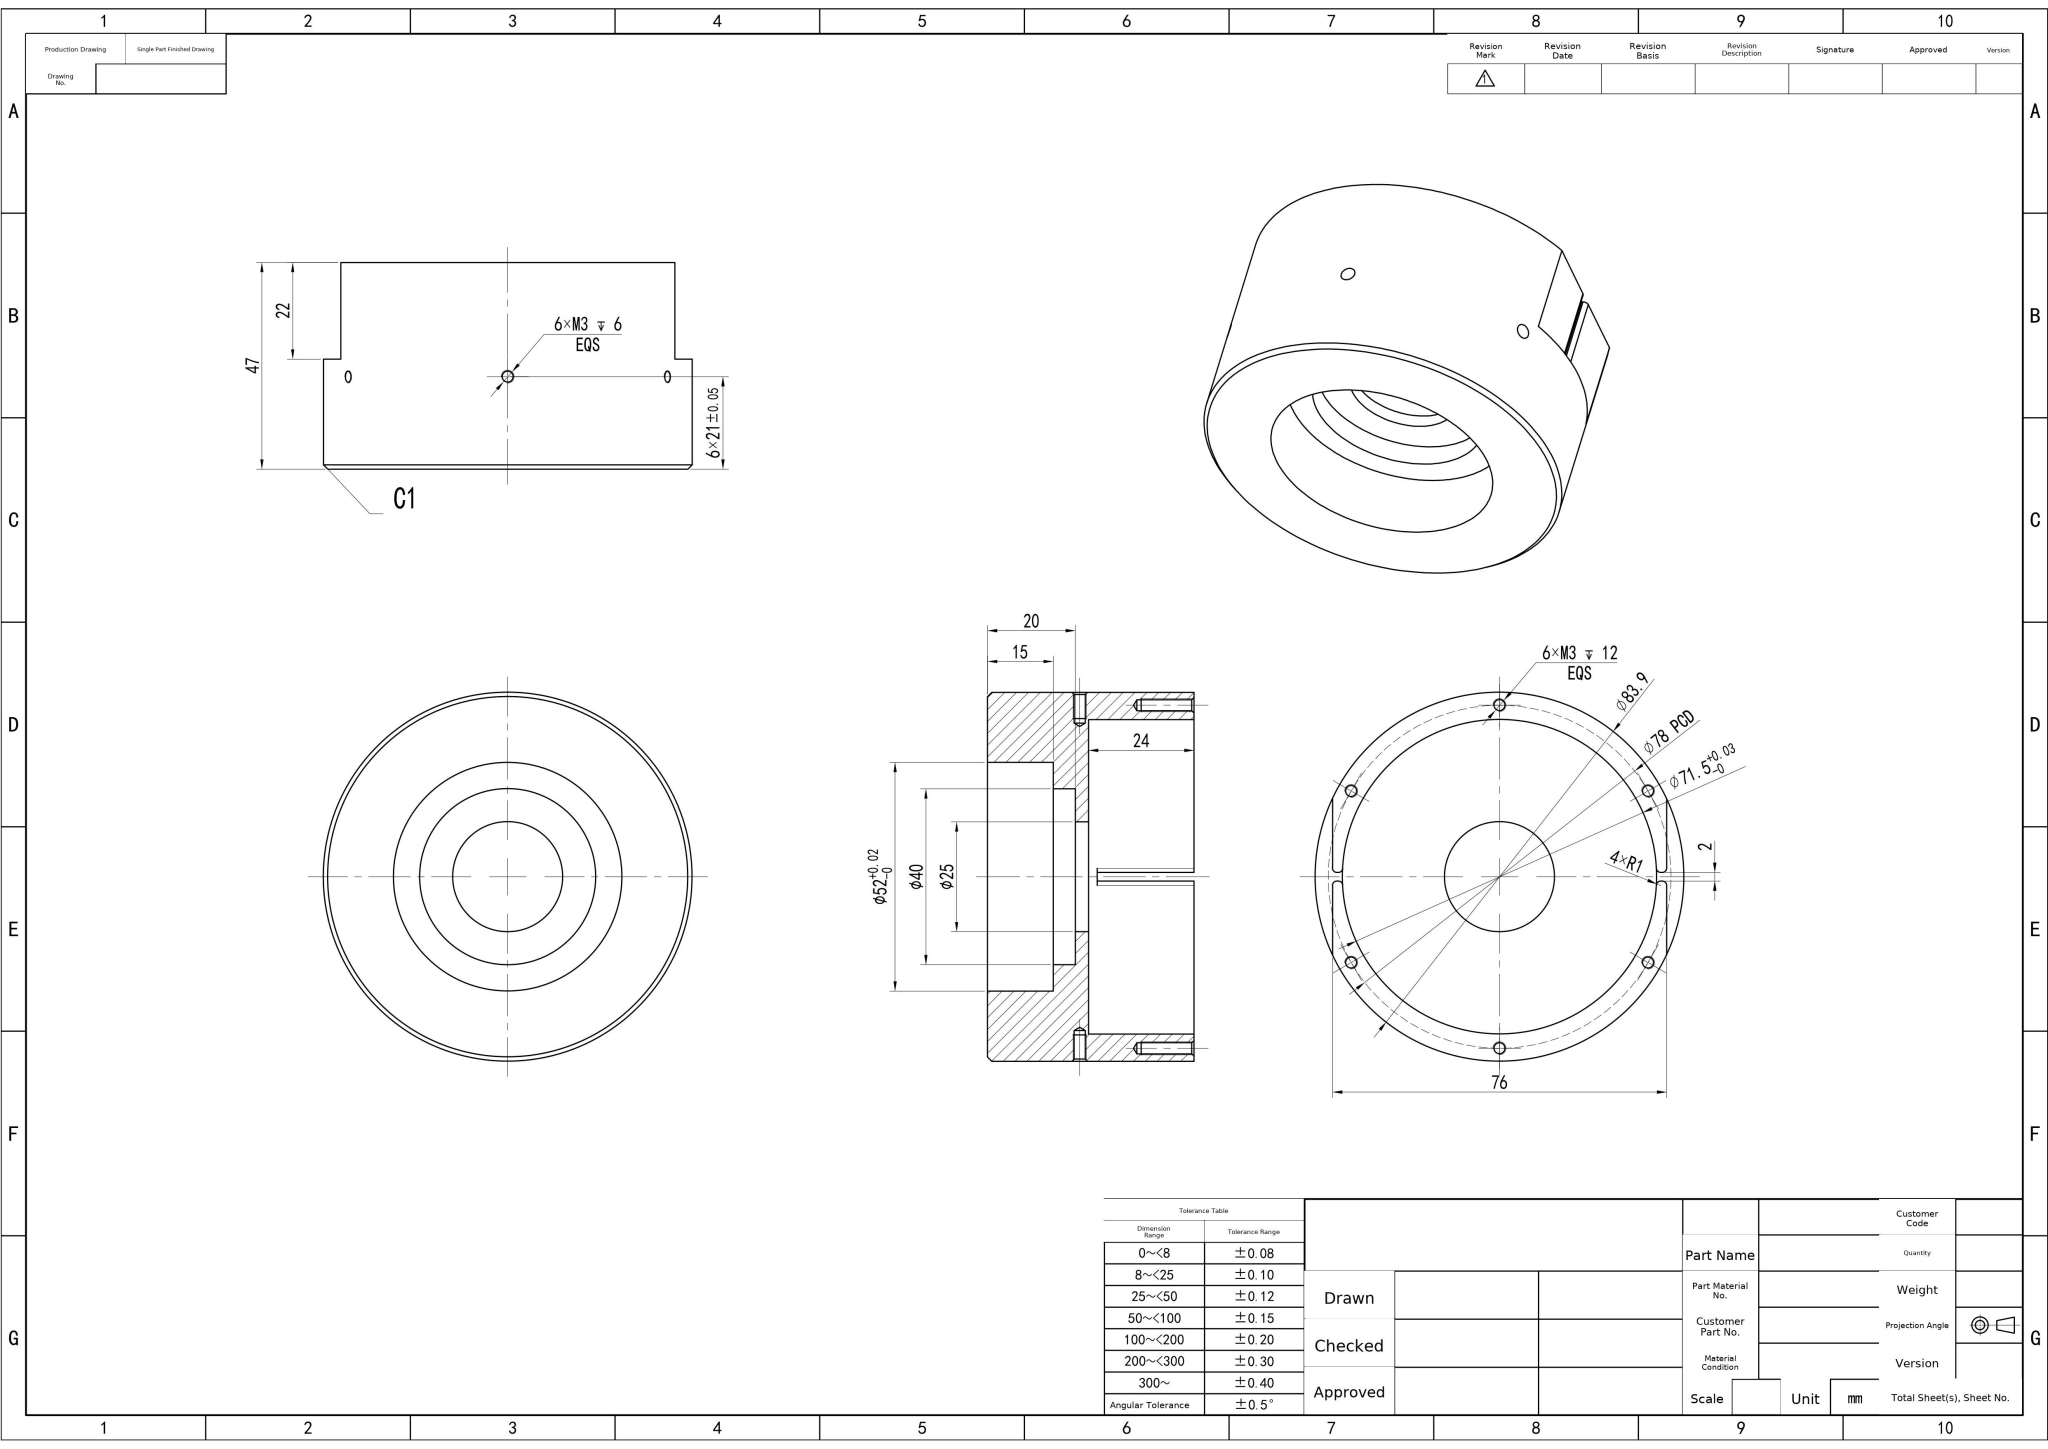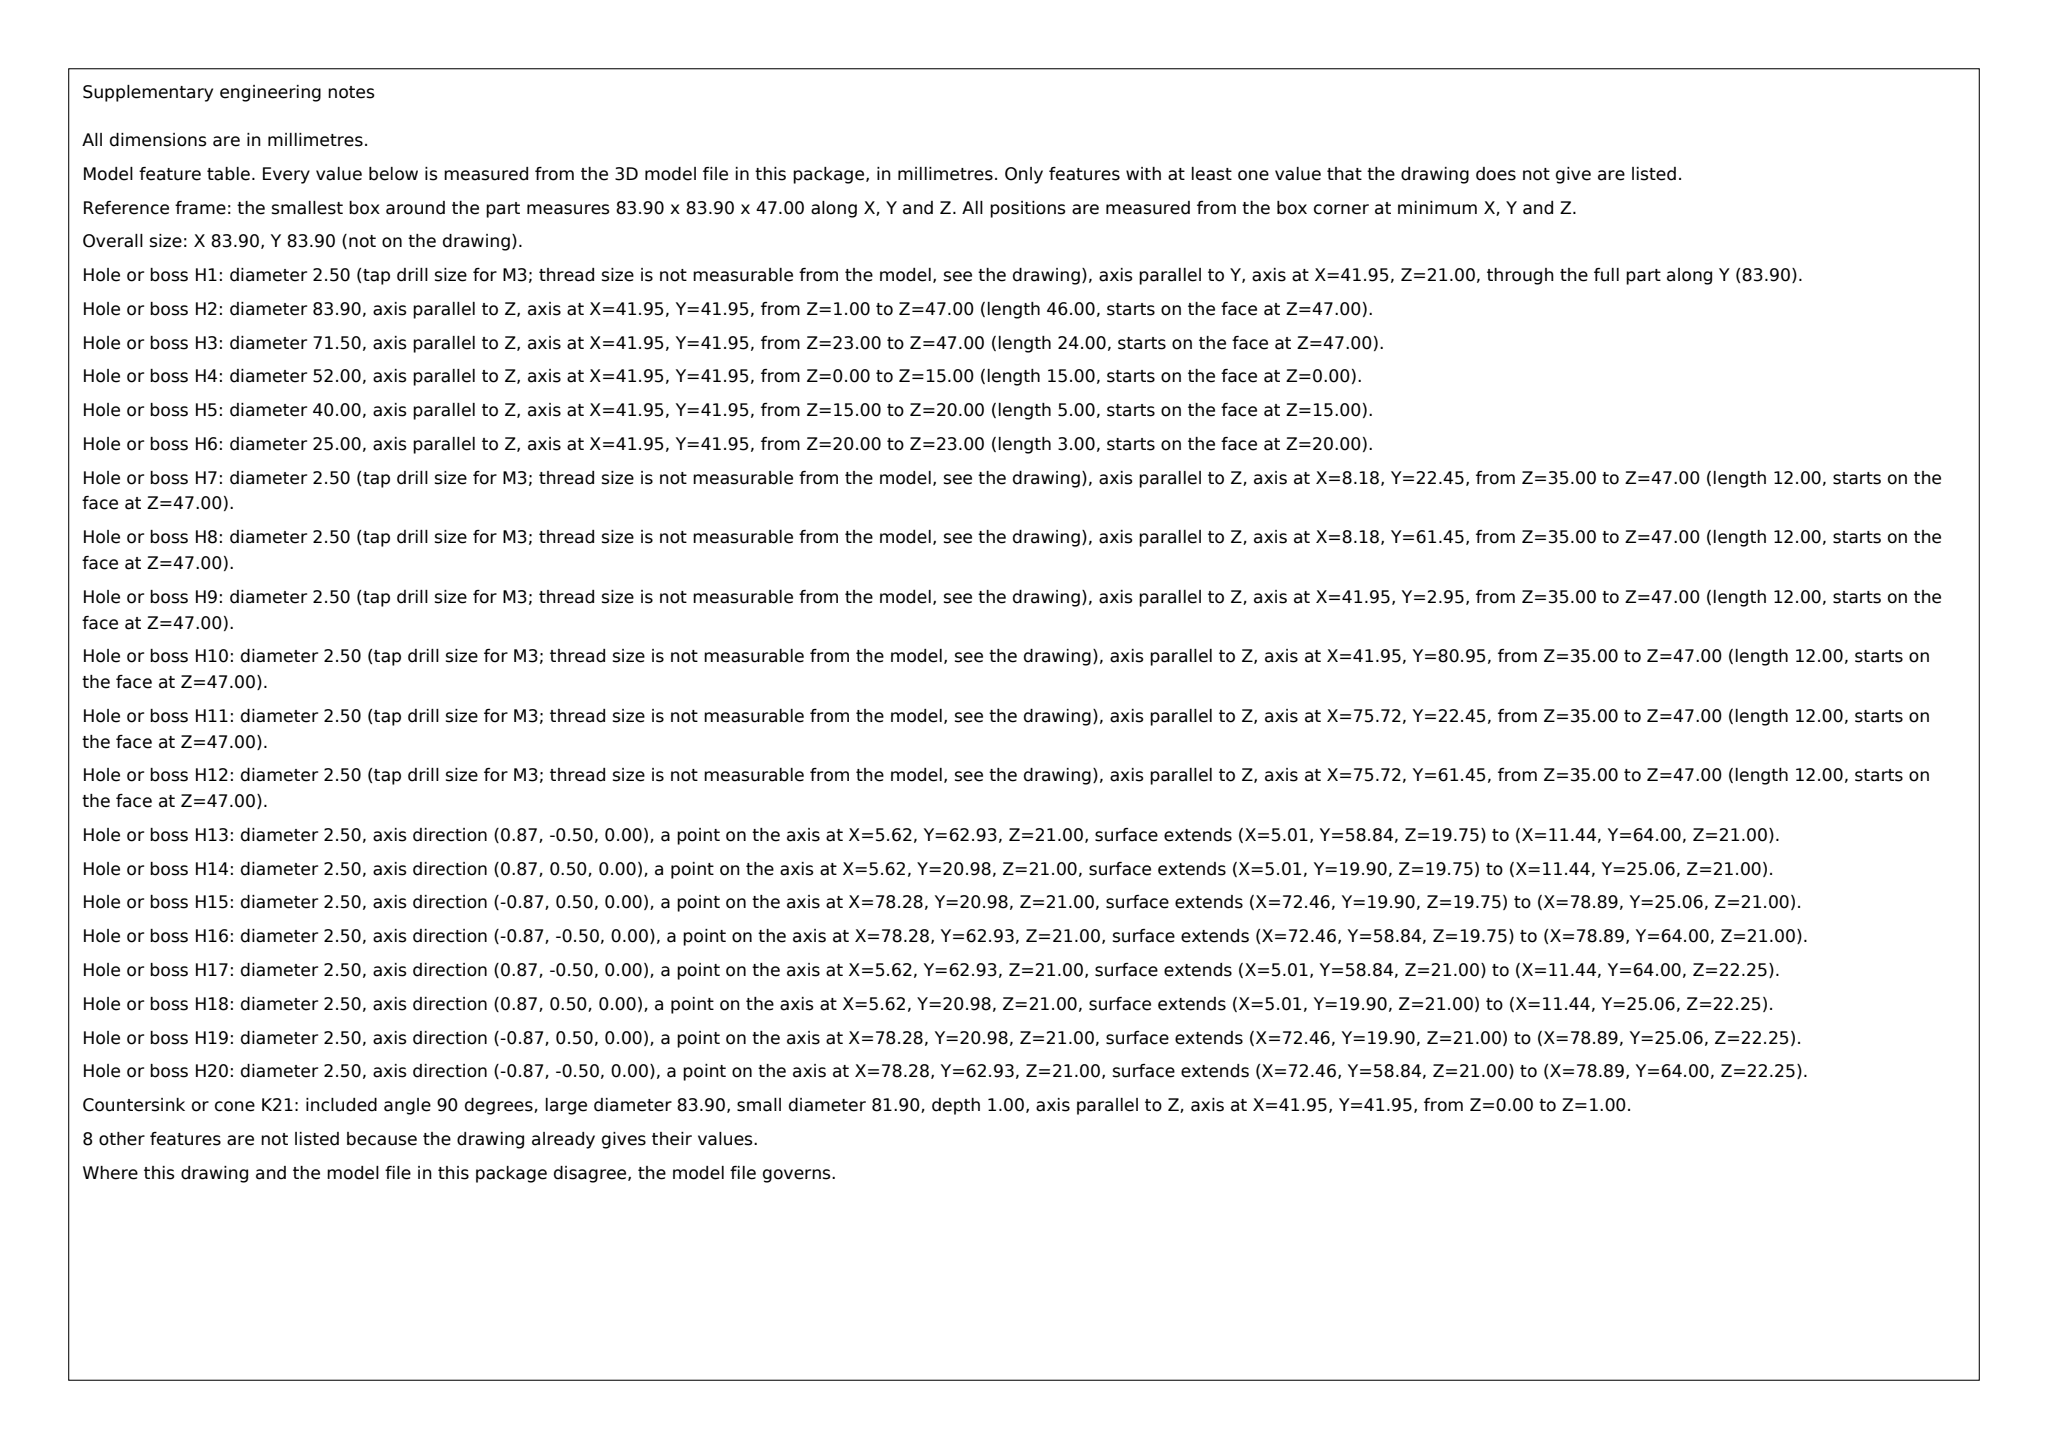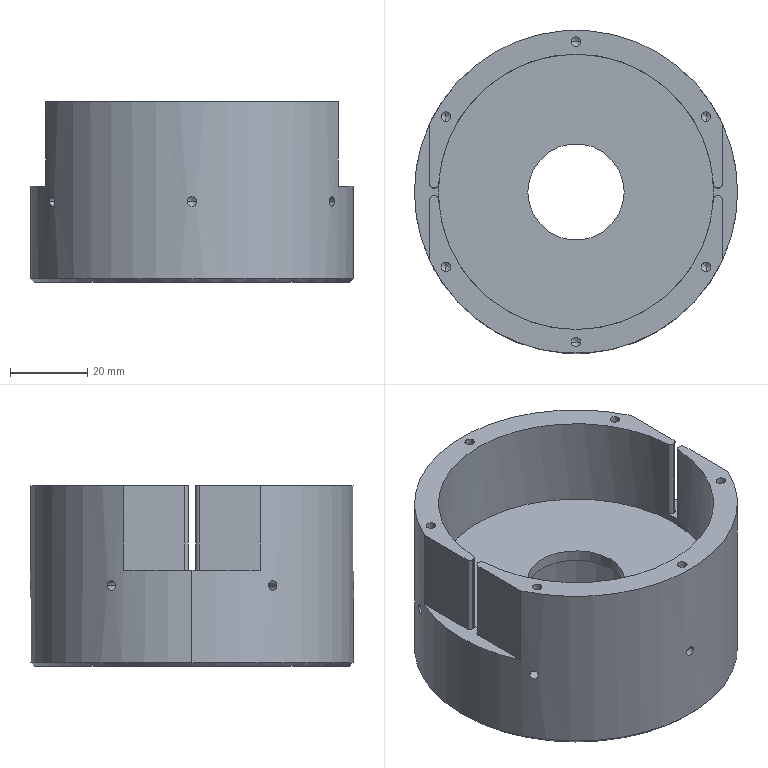Part | SolidWorks | mm | 1 solid | 84 faces | box 83.9 x 83.9 x 47 mm | volume 118800 mm3 | cylinder 42 | cone 26 | plane 16 | commonest cylinder face diameters 2.5 x24 2 x8 83.9 x2 71.5 x2 52 x2 25 x2 40 x2